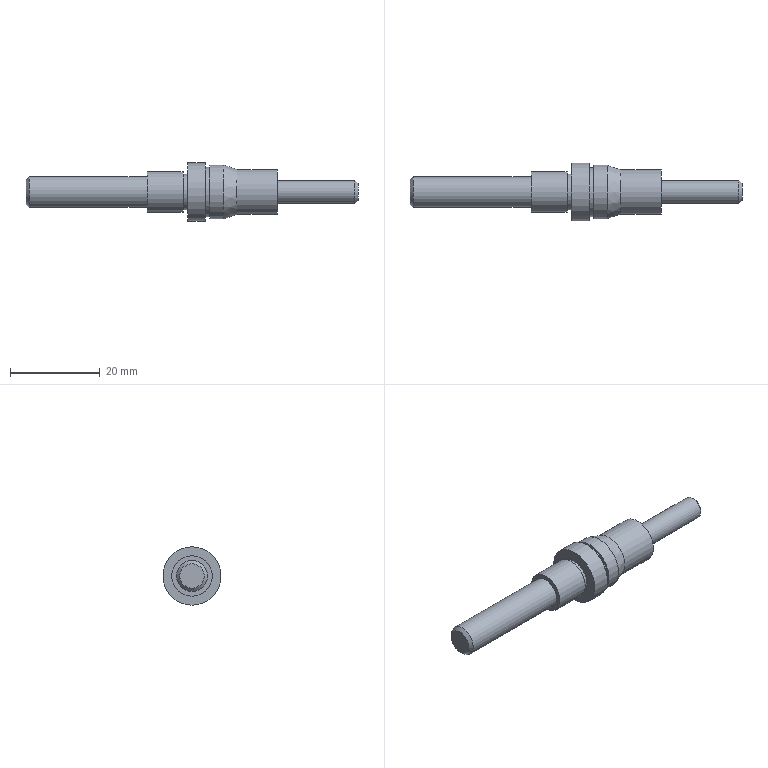Component | NX | REPL_LOC_PIN_2 | 1 solid | 19 faces | volume 3886 mm3 | plane 8 | cylinder 8 | cone 3 | commonest cylinder face diameters 6.9 x1 9 x1 8 x1 13 x1 11 x1 12 x1 10 x1 5.1 x1